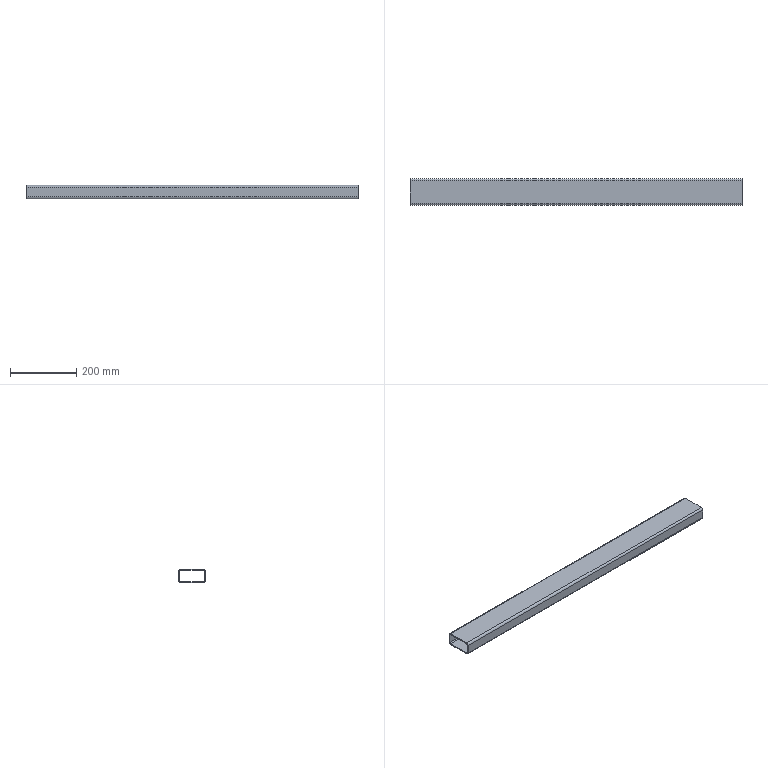Component | SolidWorks | VerticalMovingRectangularTubeWeldment-1_VerticalMovingRectangularTube-1 | 1 solid | 34 faces | volume 659617 mm3 | cylinder 24 | plane 10 | commonest cylinder face diameters 8 x16 12 x4 6 x4 | material Plain Carbon Steel